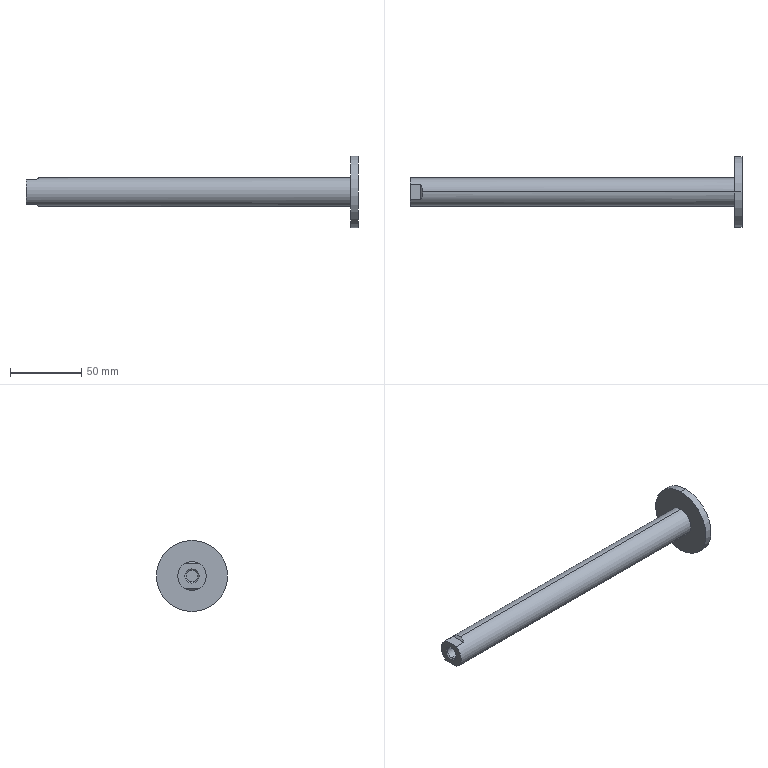Component | SolidWorks | CQ2A50-200DCZ(0_0_0)-1_CQ2A50-200DCZ(0_0_0)2-1 | 1 solid | 16 faces | box 233 x 50 x 50 mm | volume 80437 mm3 | plane 8 | cylinder 6 | cone 2 | commonest cylinder face diameters 20 x2 50 x2 8.376 x2
STEP:
#1=CARTESIAN_POINT('',(10.531,24.241,-74.524));
#2=VERTEX_POINT('',#1);
#3=CARTESIAN_POINT('',(10.59,24.034,-74.465));
#4=VERTEX_POINT('',#3);
#5=CARTESIAN_POINT('',(10.531,24.241,-74.524));
#6=CARTESIAN_POINT('',(10.57,24.178,-74.485));
#7=CARTESIAN_POINT('',(10.59,24.107,-74.465));
#8=CARTESIAN_POINT('',(10.59,24.034,-74.465));
#9=(BOUNDED_CURVE()B_SPLINE_CURVE(3,(#5,#6,#7,#8),.UNSPECIFIED.,.F.,.T.)B_SPLINE_CURVE_WITH_KNOTS((4,4),(5.728,6.283),.UNSPECIFIED.)CURVE()GEOMETRIC_REPRESENTATION_ITEM()RATIONAL_B_SPLINE_CURVE((1.,0.9745,0.9745,1.))REPRESENTATION_ITEM(''));
#10=EDGE_CURVE('',#2,#4,#9,.T.);
#11=ORIENTED_EDGE('',*,*,#10,.T.);
#12=CARTESIAN_POINT('',(19.212,24.034,-74.465));
#13=VERTEX_POINT('',#12);
#14=CARTESIAN_POINT('',(14.724,24.034,-74.465));
#15=DIRECTION('',(1.,0.,0.));
#16=VECTOR('',#15,39.37);
#17=LINE('',#14,#16);
#18=EDGE_CURVE('',#4,#13,#17,.T.);
#19=ORIENTED_EDGE('',*,*,#18,.T.);
#20=CARTESIAN_POINT('',(19.212,24.034,-75.252));
#21=VERTEX_POINT('',#20);
#22=CARTESIAN_POINT('',(19.212,24.034,-74.858));
#23=DIRECTION('',(-1.,0.,0.));
#24=DIRECTION('',(0.,0.,-1.));
#25=AXIS2_PLACEMENT_3D('',#22,#23,#24);
#26=CIRCLE('',#25,0.3937);
#27=EDGE_CURVE('',#13,#21,#26,.T.);
#28=ORIENTED_EDGE('',*,*,#27,.T.);
#29=CARTESIAN_POINT('',(10.59,24.034,-75.252));
#30=VERTEX_POINT('',#29);
#31=CARTESIAN_POINT('',(14.724,24.034,-75.252));
#32=DIRECTION('',(1.,0.,0.));
#33=VECTOR('',#32,39.37);
#34=LINE('',#31,#33);
#35=EDGE_CURVE('',#30,#21,#34,.T.);
#36=ORIENTED_EDGE('',*,*,#35,.F.);
#37=CARTESIAN_POINT('',(10.531,24.241,-75.193));
#38=VERTEX_POINT('',#37);
#39=CARTESIAN_POINT('',(10.59,24.034,-75.252));
#40=CARTESIAN_POINT('',(10.59,24.107,-75.252));
#41=CARTESIAN_POINT('',(10.57,24.178,-75.232));
#42=CARTESIAN_POINT('',(10.531,24.241,-75.193));
#43=(BOUNDED_CURVE()B_SPLINE_CURVE(3,(#39,#40,#41,#42),.UNSPECIFIED.,.F.,.T.)B_SPLINE_CURVE_WITH_KNOTS((4,4),(0.,0.5548),.UNSPECIFIED.)CURVE()GEOMETRIC_REPRESENTATION_ITEM()RATIONAL_B_SPLINE_CURVE((1.,0.9745,0.9745,1.))REPRESENTATION_ITEM(''));
#44=EDGE_CURVE('',#30,#38,#43,.T.);
#45=ORIENTED_EDGE('',*,*,#44,.T.);
#46=CARTESIAN_POINT('',(10.236,24.241,-75.193));
#47=VERTEX_POINT('',#46);
#48=CARTESIAN_POINT('',(14.724,24.241,-75.193));
#49=DIRECTION('',(-1.,0.,0.));
#50=VECTOR('',#49,39.37);
#51=LINE('',#48,#50);
#52=EDGE_CURVE('',#38,#47,#51,.T.);
#53=ORIENTED_EDGE('',*,*,#52,.T.);
#54=CARTESIAN_POINT('',(10.236,24.241,-74.524));
#55=VERTEX_POINT('',#54);
#56=CARTESIAN_POINT('',(10.236,24.034,-74.858));
#57=DIRECTION('',(1.,0.,0.));
#58=DIRECTION('',(0.,0.,-1.));
#59=AXIS2_PLACEMENT_3D('',#56,#57,#58);
#60=CIRCLE('',#59,0.3937);
#61=EDGE_CURVE('',#47,#55,#60,.T.);
#62=ORIENTED_EDGE('',*,*,#61,.T.);
#63=CARTESIAN_POINT('',(14.724,24.241,-74.524));
#64=DIRECTION('',(1.,0.,0.));
#65=VECTOR('',#64,39.37);
#66=LINE('',#63,#65);
#67=EDGE_CURVE('',#55,#2,#66,.T.);
#68=ORIENTED_EDGE('',*,*,#67,.T.);
#69=EDGE_LOOP('',(#11,#19,#28,#36,#45,#53,#62,#68));
#70=FACE_OUTER_BOUND('',#69,.T.);
#71=CARTESIAN_POINT('',(14.724,24.034,-74.858));
#72=DIRECTION('',(1.,0.,0.));
#73=DIRECTION('',(0.,0.,-1.));
#74=AXIS2_PLACEMENT_3D('',#71,#72,#73);
#75=CYLINDRICAL_SURFACE('',#74,0.3937);
#76=ADVANCED_FACE('',(#70),#75,.T.);
#77=CARTESIAN_POINT('',(19.212,24.034,-73.874));
#78=VERTEX_POINT('',#77);
#79=CARTESIAN_POINT('',(19.212,24.034,-75.843));
#80=VERTEX_POINT('',#79);
#81=CARTESIAN_POINT('',(19.212,24.034,-74.858));
#82=DIRECTION('',(-1.,0.,0.));
#83=DIRECTION('',(0.,0.,-1.));
#84=AXIS2_PLACEMENT_3D('',#81,#82,#83);
#85=CIRCLE('',#84,0.9843);
#86=EDGE_CURVE('',#78,#80,#85,.T.);
#87=ORIENTED_EDGE('',*,*,#86,.F.);
#88=CARTESIAN_POINT('',(19.409,24.034,-73.874));
#89=VERTEX_POINT('',#88);
#90=CARTESIAN_POINT('',(19.311,24.034,-73.874));
#91=DIRECTION('',(1.,0.,0.));
#92=VECTOR('',#91,39.37);
#93=LINE('',#90,#92);
#94=EDGE_CURVE('',#78,#89,#93,.T.);
#95=ORIENTED_EDGE('',*,*,#94,.T.);
#96=CARTESIAN_POINT('',(19.409,24.034,-75.843));
#97=VERTEX_POINT('',#96);
#98=CARTESIAN_POINT('',(19.409,24.034,-74.858));
#99=DIRECTION('',(-1.,0.,0.));
#100=DIRECTION('',(0.,0.,-1.));
#101=AXIS2_PLACEMENT_3D('',#98,#99,#100);
#102=CIRCLE('',#101,0.9843);
#103=EDGE_CURVE('',#89,#97,#102,.T.);
#104=ORIENTED_EDGE('',*,*,#103,.T.);
#105=CARTESIAN_POINT('',(19.311,24.034,-75.843));
#106=DIRECTION('',(1.,0.,0.));
#107=VECTOR('',#106,39.37);
#108=LINE('',#105,#107);
#109=EDGE_CURVE('',#80,#97,#108,.T.);
#110=ORIENTED_EDGE('',*,*,#109,.F.);
#111=EDGE_LOOP('',(#87,#95,#104,#110));
#112=FACE_OUTER_BOUND('',#111,.T.);
#113=CARTESIAN_POINT('',(19.311,24.034,-74.858));
#114=DIRECTION('',(1.,0.,0.));
#115=DIRECTION('',(0.,0.,-1.));
#116=AXIS2_PLACEMENT_3D('',#113,#114,#115);
#117=CYLINDRICAL_SURFACE('',#116,0.9843);
#118=ADVANCED_FACE('',(#112),#117,.T.);
#119=CARTESIAN_POINT('',(10.268,24.034,-75.023));
#120=VERTEX_POINT('',#119);
#121=CARTESIAN_POINT('',(10.268,24.034,-74.693));
#122=VERTEX_POINT('',#121);
#123=CARTESIAN_POINT('',(10.268,24.034,-74.858));
#124=DIRECTION('',(-1.,0.,0.));
#125=DIRECTION('',(0.,1.,0.));
#126=AXIS2_PLACEMENT_3D('',#123,#124,#125);
#127=CIRCLE('',#126,0.1649);
#128=EDGE_CURVE('',#120,#122,#127,.T.);
#129=ORIENTED_EDGE('',*,*,#128,.F.);
#130=CARTESIAN_POINT('',(10.236,24.034,-75.055));
#131=VERTEX_POINT('',#130);
#132=CARTESIAN_POINT('',(10.236,24.034,-75.055));
#133=DIRECTION('',(-0.7071,0.,-0.7071));
#134=VECTOR('',#133,39.37);
#135=LINE('',#132,#134);
#136=EDGE_CURVE('',#120,#131,#135,.T.);
#137=ORIENTED_EDGE('',*,*,#136,.T.);
#138=CARTESIAN_POINT('',(10.236,24.034,-74.661));
#139=VERTEX_POINT('',#138);
#140=CARTESIAN_POINT('',(10.236,24.034,-74.858));
#141=DIRECTION('',(1.,0.,0.));
#142=DIRECTION('',(0.,0.,1.));
#143=AXIS2_PLACEMENT_3D('',#140,#141,#142);
#144=CIRCLE('',#143,0.1969);
#145=EDGE_CURVE('',#139,#131,#144,.T.);
#146=ORIENTED_EDGE('',*,*,#145,.F.);
#147=CARTESIAN_POINT('',(10.236,24.034,-74.661));
#148=DIRECTION('',(-0.7071,0.,0.7071));
#149=VECTOR('',#148,39.37);
#150=LINE('',#147,#149);
#151=EDGE_CURVE('',#122,#139,#150,.T.);
#152=ORIENTED_EDGE('',*,*,#151,.F.);
#153=EDGE_LOOP('',(#129,#137,#146,#152));
#154=FACE_OUTER_BOUND('',#153,.T.);
#155=CARTESIAN_POINT('',(10.236,24.034,-74.858));
#156=DIRECTION('',(-1.,0.,0.));
#157=DIRECTION('',(0.,0.,1.));
#158=AXIS2_PLACEMENT_3D('',#155,#156,#157);
#159=CONICAL_SURFACE('',#158,0.1969,0.7854);
#160=ADVANCED_FACE('',(#154),#159,.F.);
#161=ORIENTED_EDGE('',*,*,#128,.T.);
#162=CARTESIAN_POINT('',(10.827,24.034,-74.693));
#163=VERTEX_POINT('',#162);
#164=CARTESIAN_POINT('',(10.547,24.034,-74.693));
#165=DIRECTION('',(1.,0.,0.));
#166=VECTOR('',#165,39.37);
#167=LINE('',#164,#166);
#168=EDGE_CURVE('',#122,#163,#167,.T.);
#169=ORIENTED_EDGE('',*,*,#168,.T.);
#170=CARTESIAN_POINT('',(10.827,24.034,-75.023));
#171=VERTEX_POINT('',#170);
#172=CARTESIAN_POINT('',(10.827,24.034,-74.858));
#173=DIRECTION('',(-1.,0.,0.));
#174=DIRECTION('',(0.,0.,-1.));
#175=AXIS2_PLACEMENT_3D('',#172,#173,#174);
#176=CIRCLE('',#175,0.1649);
#177=EDGE_CURVE('',#171,#163,#176,.T.);
#178=ORIENTED_EDGE('',*,*,#177,.F.);
#179=CARTESIAN_POINT('',(10.547,24.034,-75.023));
#180=DIRECTION('',(1.,0.,0.));
#181=VECTOR('',#180,39.37);
#182=LINE('',#179,#181);
#183=EDGE_CURVE('',#120,#171,#182,.T.);
#184=ORIENTED_EDGE('',*,*,#183,.F.);
#185=EDGE_LOOP('',(#161,#169,#178,#184));
#186=FACE_OUTER_BOUND('',#185,.T.);
#187=CARTESIAN_POINT('',(10.547,24.034,-74.858));
#188=DIRECTION('',(1.,0.,0.));
#189=DIRECTION('',(0.,0.,-1.));
#190=AXIS2_PLACEMENT_3D('',#187,#188,#189);
#191=CYLINDRICAL_SURFACE('',#190,0.1649);
#192=ADVANCED_FACE('',(#186),#191,.F.);
#193=ORIENTED_EDGE('',*,*,#18,.F.);
#194=CARTESIAN_POINT('',(10.531,23.826,-74.524));
#195=VERTEX_POINT('',#194);
#196=CARTESIAN_POINT('',(10.59,24.034,-74.465));
#197=CARTESIAN_POINT('',(10.59,23.96,-74.465));
#198=CARTESIAN_POINT('',(10.57,23.889,-74.485));
#199=CARTESIAN_POINT('',(10.531,23.826,-74.524));
#200=(BOUNDED_CURVE()B_SPLINE_CURVE(3,(#196,#197,#198,#199),.UNSPECIFIED.,.F.,.F.)B_SPLINE_CURVE_WITH_KNOTS((4,4),(0.,0.5548),.UNSPECIFIED.)CURVE()GEOMETRIC_REPRESENTATION_ITEM()RATIONAL_B_SPLINE_CURVE((1.,0.9745,0.9745,1.))REPRESENTATION_ITEM(''));
#201=EDGE_CURVE('',#4,#195,#200,.T.);
#202=ORIENTED_EDGE('',*,*,#201,.T.);
#203=CARTESIAN_POINT('',(10.236,23.826,-74.524));
#204=VERTEX_POINT('',#203);
#205=CARTESIAN_POINT('',(14.724,23.826,-74.524));
#206=DIRECTION('',(-1.,0.,0.));
#207=VECTOR('',#206,39.37);
#208=LINE('',#205,#207);
#209=EDGE_CURVE('',#195,#204,#208,.T.);
#210=ORIENTED_EDGE('',*,*,#209,.T.);
#211=CARTESIAN_POINT('',(10.236,23.826,-75.193));
#212=VERTEX_POINT('',#211);
#213=CARTESIAN_POINT('',(10.236,24.034,-74.858));
#214=DIRECTION('',(1.,0.,0.));
#215=DIRECTION('',(0.,0.,-1.));
#216=AXIS2_PLACEMENT_3D('',#213,#214,#215);
#217=CIRCLE('',#216,0.3937);
#218=EDGE_CURVE('',#204,#212,#217,.T.);
#219=ORIENTED_EDGE('',*,*,#218,.T.);
#220=CARTESIAN_POINT('',(10.531,23.826,-75.193));
#221=VERTEX_POINT('',#220);
#222=CARTESIAN_POINT('',(14.724,23.826,-75.193));
#223=DIRECTION('',(1.,0.,0.));
#224=VECTOR('',#223,39.37);
#225=LINE('',#222,#224);
#226=EDGE_CURVE('',#212,#221,#225,.T.);
#227=ORIENTED_EDGE('',*,*,#226,.T.);
#228=CARTESIAN_POINT('',(10.531,23.826,-75.193));
#229=CARTESIAN_POINT('',(10.57,23.889,-75.232));
#230=CARTESIAN_POINT('',(10.59,23.96,-75.252));
#231=CARTESIAN_POINT('',(10.59,24.034,-75.252));
#232=(BOUNDED_CURVE()B_SPLINE_CURVE(3,(#228,#229,#230,#231),.UNSPECIFIED.,.F.,.T.)B_SPLINE_CURVE_WITH_KNOTS((4,4),(5.728,6.283),.UNSPECIFIED.)CURVE()GEOMETRIC_REPRESENTATION_ITEM()RATIONAL_B_SPLINE_CURVE((1.,0.9745,0.9745,1.))REPRESENTATION_ITEM(''));
#233=EDGE_CURVE('',#221,#30,#232,.T.);
#234=ORIENTED_EDGE('',*,*,#233,.T.);
#235=ORIENTED_EDGE('',*,*,#35,.T.);
#236=CARTESIAN_POINT('',(19.212,24.034,-74.858));
#237=DIRECTION('',(-1.,0.,0.));
#238=DIRECTION('',(0.,0.,-1.));
#239=AXIS2_PLACEMENT_3D('',#236,#237,#238);
#240=CIRCLE('',#239,0.3937);
#241=EDGE_CURVE('',#21,#13,#240,.T.);
#242=ORIENTED_EDGE('',*,*,#241,.T.);
#243=EDGE_LOOP('',(#193,#202,#210,#219,#227,#234,#235,#242));
#244=FACE_OUTER_BOUND('',#243,.T.);
#245=CARTESIAN_POINT('',(14.724,24.034,-74.858));
#246=DIRECTION('',(1.,0.,0.));
#247=DIRECTION('',(0.,0.,-1.));
#248=AXIS2_PLACEMENT_3D('',#245,#246,#247);
#249=CYLINDRICAL_SURFACE('',#248,0.3937);
#250=ADVANCED_FACE('',(#244),#249,.T.);
#251=CARTESIAN_POINT('',(19.212,24.034,-74.858));
#252=DIRECTION('',(-1.,0.,0.));
#253=DIRECTION('',(0.,0.,-1.));
#254=AXIS2_PLACEMENT_3D('',#251,#252,#253);
#255=CIRCLE('',#254,0.9843);
#256=EDGE_CURVE('',#80,#78,#255,.T.);
#257=ORIENTED_EDGE('',*,*,#256,.T.);
#258=ORIENTED_EDGE('',*,*,#86,.T.);
#259=EDGE_LOOP('',(#257,#258));
#260=FACE_OUTER_BOUND('',#259,.T.);
#261=ORIENTED_EDGE('',*,*,#241,.F.);
#262=ORIENTED_EDGE('',*,*,#27,.F.);
#263=EDGE_LOOP('',(#261,#262));
#264=FACE_BOUND('',#263,.T.);
#265=CARTESIAN_POINT('',(19.212,24.723,-74.858));
#266=DIRECTION('',(-1.,0.,0.));
#267=DIRECTION('',(0.,0.,1.));
#268=AXIS2_PLACEMENT_3D('',#265,#266,#267);
#269=PLANE('',#268);
#270=ADVANCED_FACE('',(#260,#264),#269,.T.);
#271=CARTESIAN_POINT('',(10.236,24.329,-75.193));
#272=DIRECTION('',(0.,-1.,0.));
#273=VECTOR('',#272,39.37);
#274=LINE('',#271,#273);
#275=EDGE_CURVE('',#47,#212,#274,.T.);
#276=ORIENTED_EDGE('',*,*,#275,.T.);
#277=ORIENTED_EDGE('',*,*,#218,.F.);
#278=CARTESIAN_POINT('',(10.236,24.329,-74.524));
#279=DIRECTION('',(0.,1.,0.));
#280=VECTOR('',#279,39.37);
#281=LINE('',#278,#280);
#282=EDGE_CURVE('',#204,#55,#281,.T.);
#283=ORIENTED_EDGE('',*,*,#282,.T.);
#284=ORIENTED_EDGE('',*,*,#61,.F.);
#285=EDGE_LOOP('',(#276,#277,#283,#284));
#286=FACE_OUTER_BOUND('',#285,.T.);
#287=ORIENTED_EDGE('',*,*,#145,.T.);
#288=CARTESIAN_POINT('',(10.236,24.034,-74.858));
#289=DIRECTION('',(1.,0.,0.));
#290=DIRECTION('',(0.,0.,1.));
#291=AXIS2_PLACEMENT_3D('',#288,#289,#290);
#292=CIRCLE('',#291,0.1969);
#293=EDGE_CURVE('',#131,#139,#292,.T.);
#294=ORIENTED_EDGE('',*,*,#293,.T.);
#295=EDGE_LOOP('',(#287,#294));
#296=FACE_BOUND('',#295,.T.);
#297=CARTESIAN_POINT('',(10.236,24.329,-74.858));
#298=DIRECTION('',(-1.,0.,0.));
#299=DIRECTION('',(0.,0.,1.));
#300=AXIS2_PLACEMENT_3D('',#297,#298,#299);
#301=PLANE('',#300);
#302=ADVANCED_FACE('',(#286,#296),#301,.T.);
#303=CARTESIAN_POINT('',(10.531,24.821,-74.524));
#304=DIRECTION('',(0.,-1.,0.));
#305=VECTOR('',#304,39.37);
#306=LINE('',#303,#305);
#307=EDGE_CURVE('',#2,#195,#306,.T.);
#308=ORIENTED_EDGE('',*,*,#307,.F.);
#309=ORIENTED_EDGE('',*,*,#67,.F.);
#310=ORIENTED_EDGE('',*,*,#282,.F.);
#311=ORIENTED_EDGE('',*,*,#209,.F.);
#312=EDGE_LOOP('',(#308,#309,#310,#311));
#313=FACE_OUTER_BOUND('',#312,.T.);
#314=CARTESIAN_POINT('',(10.531,24.821,-74.524));
#315=DIRECTION('',(0.,0.,-1.));
#316=DIRECTION('',(-1.,0.,0.));
#317=AXIS2_PLACEMENT_3D('',#314,#315,#316);
#318=PLANE('',#317);
#319=ADVANCED_FACE('',(#313),#318,.F.);
#320=ORIENTED_EDGE('',*,*,#307,.T.);
#321=ORIENTED_EDGE('',*,*,#201,.F.);
#322=ORIENTED_EDGE('',*,*,#10,.F.);
#323=EDGE_LOOP('',(#320,#321,#322));
#324=FACE_OUTER_BOUND('',#323,.T.);
#325=CARTESIAN_POINT('',(10.728,24.821,-74.327));
#326=DIRECTION('',(0.7071,0.,-0.7071));
#327=DIRECTION('',(-0.7071,0.,-0.7071));
#328=AXIS2_PLACEMENT_3D('',#325,#326,#327);
#329=PLANE('',#328);
#330=ADVANCED_FACE('',(#324),#329,.F.);
#331=ORIENTED_EDGE('',*,*,#94,.F.);
#332=ORIENTED_EDGE('',*,*,#256,.F.);
#333=ORIENTED_EDGE('',*,*,#109,.T.);
#334=CARTESIAN_POINT('',(19.409,24.034,-74.858));
#335=DIRECTION('',(-1.,0.,0.));
#336=DIRECTION('',(0.,0.,-1.));
#337=AXIS2_PLACEMENT_3D('',#334,#335,#336);
#338=CIRCLE('',#337,0.9843);
#339=EDGE_CURVE('',#97,#89,#338,.T.);
#340=ORIENTED_EDGE('',*,*,#339,.T.);
#341=EDGE_LOOP('',(#331,#332,#333,#340));
#342=FACE_OUTER_BOUND('',#341,.T.);
#343=CARTESIAN_POINT('',(19.311,24.034,-74.858));
#344=DIRECTION('',(1.,0.,0.));
#345=DIRECTION('',(0.,0.,-1.));
#346=AXIS2_PLACEMENT_3D('',#343,#344,#345);
#347=CYLINDRICAL_SURFACE('',#346,0.9843);
#348=ADVANCED_FACE('',(#342),#347,.T.);
#349=ORIENTED_EDGE('',*,*,#275,.F.);
#350=ORIENTED_EDGE('',*,*,#52,.F.);
#351=CARTESIAN_POINT('',(10.531,24.821,-75.193));
#352=DIRECTION('',(0.,1.,0.));
#353=VECTOR('',#352,39.37);
#354=LINE('',#351,#353);
#355=EDGE_CURVE('',#221,#38,#354,.T.);
#356=ORIENTED_EDGE('',*,*,#355,.F.);
#357=ORIENTED_EDGE('',*,*,#226,.F.);
#358=EDGE_LOOP('',(#349,#350,#356,#357));
#359=FACE_OUTER_BOUND('',#358,.T.);
#360=CARTESIAN_POINT('',(10.236,24.821,-75.193));
#361=DIRECTION('',(0.,0.,1.));
#362=DIRECTION('',(1.,0.,-0.));
#363=AXIS2_PLACEMENT_3D('',#360,#361,#362);
#364=PLANE('',#363);
#365=ADVANCED_FACE('',(#359),#364,.F.);
#366=ORIENTED_EDGE('',*,*,#355,.T.);
#367=ORIENTED_EDGE('',*,*,#44,.F.);
#368=ORIENTED_EDGE('',*,*,#233,.F.);
#369=EDGE_LOOP('',(#366,#367,#368));
#370=FACE_OUTER_BOUND('',#369,.T.);
#371=CARTESIAN_POINT('',(10.531,24.821,-75.193));
#372=DIRECTION('',(0.7071,0.,0.7071));
#373=DIRECTION('',(0.7071,0.,-0.7071));
#374=AXIS2_PLACEMENT_3D('',#371,#372,#373);
#375=PLANE('',#374);
#376=ADVANCED_FACE('',(#370),#375,.F.);
#377=ORIENTED_EDGE('',*,*,#136,.F.);
#378=CARTESIAN_POINT('',(10.268,24.034,-74.858));
#379=DIRECTION('',(-1.,0.,0.));
#380=DIRECTION('',(0.,1.,0.));
#381=AXIS2_PLACEMENT_3D('',#378,#379,#380);
#382=CIRCLE('',#381,0.1649);
#383=EDGE_CURVE('',#122,#120,#382,.T.);
#384=ORIENTED_EDGE('',*,*,#383,.F.);
#385=ORIENTED_EDGE('',*,*,#151,.T.);
#386=ORIENTED_EDGE('',*,*,#293,.F.);
#387=EDGE_LOOP('',(#377,#384,#385,#386));
#388=FACE_OUTER_BOUND('',#387,.T.);
#389=CARTESIAN_POINT('',(10.236,24.034,-74.858));
#390=DIRECTION('',(-1.,0.,0.));
#391=DIRECTION('',(0.,0.,1.));
#392=AXIS2_PLACEMENT_3D('',#389,#390,#391);
#393=CONICAL_SURFACE('',#392,0.1969,0.7854);
#394=ADVANCED_FACE('',(#388),#393,.F.);
#395=ORIENTED_EDGE('',*,*,#339,.F.);
#396=ORIENTED_EDGE('',*,*,#103,.F.);
#397=EDGE_LOOP('',(#395,#396));
#398=FACE_OUTER_BOUND('',#397,.T.);
#399=CARTESIAN_POINT('',(19.409,24.526,-74.858));
#400=DIRECTION('',(1.,0.,0.));
#401=DIRECTION('',(0.,0.,-1.));
#402=AXIS2_PLACEMENT_3D('',#399,#400,#401);
#403=PLANE('',#402);
#404=ADVANCED_FACE('',(#398),#403,.T.);
#405=ORIENTED_EDGE('',*,*,#168,.F.);
#406=ORIENTED_EDGE('',*,*,#383,.T.);
#407=ORIENTED_EDGE('',*,*,#183,.T.);
#408=CARTESIAN_POINT('',(10.827,24.034,-74.858));
#409=DIRECTION('',(-1.,0.,0.));
#410=DIRECTION('',(0.,0.,-1.));
#411=AXIS2_PLACEMENT_3D('',#408,#409,#410);
#412=CIRCLE('',#411,0.1649);
#413=EDGE_CURVE('',#163,#171,#412,.T.);
#414=ORIENTED_EDGE('',*,*,#413,.F.);
#415=EDGE_LOOP('',(#405,#406,#407,#414));
#416=FACE_OUTER_BOUND('',#415,.T.);
#417=CARTESIAN_POINT('',(10.547,24.034,-74.858));
#418=DIRECTION('',(1.,0.,0.));
#419=DIRECTION('',(0.,0.,-1.));
#420=AXIS2_PLACEMENT_3D('',#417,#418,#419);
#421=CYLINDRICAL_SURFACE('',#420,0.1649);
#422=ADVANCED_FACE('',(#416),#421,.F.);
#423=ORIENTED_EDGE('',*,*,#177,.T.);
#424=ORIENTED_EDGE('',*,*,#413,.T.);
#425=EDGE_LOOP('',(#423,#424));
#426=FACE_OUTER_BOUND('',#425,.T.);
#427=CARTESIAN_POINT('',(10.827,24.116,-74.858));
#428=DIRECTION('',(-1.,-0.,0.));
#429=DIRECTION('',(0.,-1.,0.));
#430=AXIS2_PLACEMENT_3D('',#427,#428,#429);
#431=PLANE('',#430);
#432=ADVANCED_FACE('',(#426),#431,.T.);
#433=CLOSED_SHELL('',(#76,#118,#160,#192,#250,#270,#302,#319,#330,#348,#365,#376,#394,#404,#422,#432));
#434=MANIFOLD_SOLID_BREP('',#433);
#435=CARTESIAN_POINT('',(0.,0.,0.));
#436=DIRECTION('',(0.,0.,1.));
#437=DIRECTION('',(1.,0.,0.));
#438=AXIS2_PLACEMENT_3D('',#435,#436,#437);
#439=(LENGTH_UNIT()NAMED_UNIT(*)SI_UNIT($,.METRE.));
#440=LENGTH_MEASURE_WITH_UNIT(LENGTH_MEASURE(0.0254),#439);
#441=DIMENSIONAL_EXPONENTS(1.,0.,0.,0.,0.,0.,0.);
#442=(CONVERSION_BASED_UNIT('',#440)LENGTH_UNIT()NAMED_UNIT(#441));
#443=UNCERTAINTY_MEASURE_WITH_UNIT(LENGTH_MEASURE(0.00001),#442,'','');
#444=(NAMED_UNIT(*)PLANE_ANGLE_UNIT()SI_UNIT($,.RADIAN.));
#445=(NAMED_UNIT(*)SI_UNIT($,.STERADIAN.)SOLID_ANGLE_UNIT());
#446=(GEOMETRIC_REPRESENTATION_CONTEXT(3)GLOBAL_UNCERTAINTY_ASSIGNED_CONTEXT((#443))GLOBAL_UNIT_ASSIGNED_CONTEXT((#442,#444,#445))REPRESENTATION_CONTEXT('',''));
#447=ADVANCED_BREP_SHAPE_REPRESENTATION('',(#434,#438),#446);
#448=COLOUR_RGB('',0.7922,0.8196,0.9333);
#449=FILL_AREA_STYLE_COLOUR('',#448);
#450=FILL_AREA_STYLE('',(#449));
#451=SURFACE_STYLE_FILL_AREA(#450);
#452=SURFACE_SIDE_STYLE('',(#451));
#453=SURFACE_STYLE_USAGE(.BOTH.,#452);
#454=PRESENTATION_STYLE_ASSIGNMENT((#453));
#455=STYLED_ITEM('',(#454),#434);
#456=(LENGTH_UNIT()NAMED_UNIT(*)SI_UNIT($,.METRE.));
#457=LENGTH_MEASURE_WITH_UNIT(LENGTH_MEASURE(0.0254),#456);
#458=DIMENSIONAL_EXPONENTS(1.,0.,0.,0.,0.,0.,0.);
#459=(CONVERSION_BASED_UNIT('',#457)LENGTH_UNIT()NAMED_UNIT(#458));
#460=UNCERTAINTY_MEASURE_WITH_UNIT(LENGTH_MEASURE(0.00001),#459,'','');
#461=(NAMED_UNIT(*)PLANE_ANGLE_UNIT()SI_UNIT($,.RADIAN.));
#462=(NAMED_UNIT(*)SI_UNIT($,.STERADIAN.)SOLID_ANGLE_UNIT());
#463=(GEOMETRIC_REPRESENTATION_CONTEXT(3)GLOBAL_UNCERTAINTY_ASSIGNED_CONTEXT((#460))GLOBAL_UNIT_ASSIGNED_CONTEXT((#459,#461,#462))REPRESENTATION_CONTEXT('',''));
#464=MECHANICAL_DESIGN_GEOMETRIC_PRESENTATION_REPRESENTATION('',(#455),#463);
#465=PRESENTATION_LAYER_ASSIGNMENT('','',(#455));